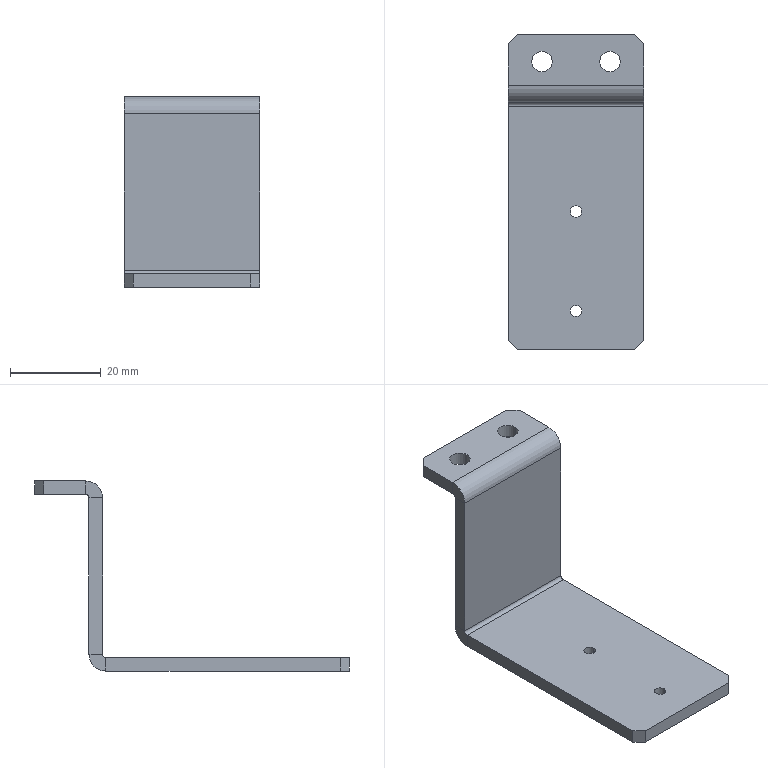Component | SolidWorks | SFTJ-07-DragChainBracket-1 | 1 solid | 34 faces | box 30 x 69.5 x 42 mm | volume 9443 mm3 | plane 22 | cylinder 12 | commonest cylinder face diameters 4.5 x4 2.5 x4 1.473 x2 7.473 x2 | material 201 Annealed Stainless Steel (SS)
STEP:
#1=COLOUR_RGB('',0.7922,0.8196,0.9333);
#2=FILL_AREA_STYLE_COLOUR('',#1);
#3=FILL_AREA_STYLE('',(#2));
#4=SURFACE_STYLE_FILL_AREA(#3);
#5=SURFACE_SIDE_STYLE('',(#4));
#6=SURFACE_STYLE_USAGE(.BOTH.,#5);
#7=PRESENTATION_STYLE_ASSIGNMENT((#6));
#8=CARTESIAN_POINT('',(-8.868,1.839,-2.615));
#9=VERTEX_POINT('',#8);
#10=CARTESIAN_POINT('',(-9.046,1.839,-2.615));
#11=VERTEX_POINT('',#10);
#12=CARTESIAN_POINT('',(-8.957,1.839,-2.615));
#13=DIRECTION('',(-0.,-0.,-1.));
#14=DIRECTION('',(-1.,0.,0.));
#15=AXIS2_PLACEMENT_3D('',#12,#13,#14);
#16=CIRCLE('',#15,0.08858);
#17=EDGE_CURVE('',#9,#11,#16,.T.);
#18=ORIENTED_EDGE('',*,*,#17,.F.);
#19=CARTESIAN_POINT('',(-8.868,1.839,-2.733));
#20=VERTEX_POINT('',#19);
#21=CARTESIAN_POINT('',(-8.868,1.839,-2.733));
#22=DIRECTION('',(-0.,-0.,-1.));
#23=VECTOR('',#22,39.37);
#24=LINE('',#21,#23);
#25=EDGE_CURVE('',#9,#20,#24,.T.);
#26=ORIENTED_EDGE('',*,*,#25,.T.);
#27=CARTESIAN_POINT('',(-9.046,1.839,-2.733));
#28=VERTEX_POINT('',#27);
#29=CARTESIAN_POINT('',(-8.957,1.839,-2.733));
#30=DIRECTION('',(-0.,-0.,-1.));
#31=DIRECTION('',(-1.,0.,0.));
#32=AXIS2_PLACEMENT_3D('',#29,#30,#31);
#33=CIRCLE('',#32,0.08858);
#34=EDGE_CURVE('',#20,#28,#33,.T.);
#35=ORIENTED_EDGE('',*,*,#34,.T.);
#36=CARTESIAN_POINT('',(-9.046,1.839,-2.733));
#37=DIRECTION('',(-0.,-0.,-1.));
#38=VECTOR('',#37,39.37);
#39=LINE('',#36,#38);
#40=EDGE_CURVE('',#11,#28,#39,.T.);
#41=ORIENTED_EDGE('',*,*,#40,.F.);
#42=EDGE_LOOP('',(#18,#26,#35,#41));
#43=FACE_OUTER_BOUND('',#42,.T.);
#44=CARTESIAN_POINT('',(-8.957,1.839,-2.733));
#45=DIRECTION('',(-0.,-0.,-1.));
#46=DIRECTION('',(-1.,0.,0.));
#47=AXIS2_PLACEMENT_3D('',#44,#45,#46);
#48=CYLINDRICAL_SURFACE('',#47,0.08858);
#49=ADVANCED_FACE('',(#43),#48,.F.);
#50=CARTESIAN_POINT('',(-9.459,1.839,-2.615));
#51=VERTEX_POINT('',#50);
#52=CARTESIAN_POINT('',(-9.636,1.839,-2.615));
#53=VERTEX_POINT('',#52);
#54=CARTESIAN_POINT('',(-9.548,1.839,-2.615));
#55=DIRECTION('',(-0.,-0.,-1.));
#56=DIRECTION('',(-1.,0.,0.));
#57=AXIS2_PLACEMENT_3D('',#54,#55,#56);
#58=CIRCLE('',#57,0.08858);
#59=EDGE_CURVE('',#51,#53,#58,.T.);
#60=ORIENTED_EDGE('',*,*,#59,.F.);
#61=CARTESIAN_POINT('',(-9.459,1.839,-2.733));
#62=VERTEX_POINT('',#61);
#63=CARTESIAN_POINT('',(-9.459,1.839,-2.733));
#64=DIRECTION('',(-0.,-0.,-1.));
#65=VECTOR('',#64,39.37);
#66=LINE('',#63,#65);
#67=EDGE_CURVE('',#51,#62,#66,.T.);
#68=ORIENTED_EDGE('',*,*,#67,.T.);
#69=CARTESIAN_POINT('',(-9.636,1.839,-2.733));
#70=VERTEX_POINT('',#69);
#71=CARTESIAN_POINT('',(-9.548,1.839,-2.733));
#72=DIRECTION('',(-0.,-0.,-1.));
#73=DIRECTION('',(-1.,0.,0.));
#74=AXIS2_PLACEMENT_3D('',#71,#72,#73);
#75=CIRCLE('',#74,0.08858);
#76=EDGE_CURVE('',#62,#70,#75,.T.);
#77=ORIENTED_EDGE('',*,*,#76,.T.);
#78=CARTESIAN_POINT('',(-9.636,1.839,-2.733));
#79=DIRECTION('',(-0.,-0.,-1.));
#80=VECTOR('',#79,39.37);
#81=LINE('',#78,#80);
#82=EDGE_CURVE('',#53,#70,#81,.T.);
#83=ORIENTED_EDGE('',*,*,#82,.F.);
#84=EDGE_LOOP('',(#60,#68,#77,#83));
#85=FACE_OUTER_BOUND('',#84,.T.);
#86=CARTESIAN_POINT('',(-9.548,1.839,-2.733));
#87=DIRECTION('',(-0.,-0.,-1.));
#88=DIRECTION('',(-1.,0.,0.));
#89=AXIS2_PLACEMENT_3D('',#86,#87,#88);
#90=CYLINDRICAL_SURFACE('',#89,0.08858);
#91=ADVANCED_FACE('',(#85),#90,.F.);
#92=CARTESIAN_POINT('',(-9.302,-0.326,-4.15));
#93=VERTEX_POINT('',#92);
#94=CARTESIAN_POINT('',(-9.203,-0.326,-4.15));
#95=VERTEX_POINT('',#94);
#96=CARTESIAN_POINT('',(-9.252,-0.326,-4.15));
#97=DIRECTION('',(0.,0.,1.));
#98=DIRECTION('',(0.,1.,0.));
#99=AXIS2_PLACEMENT_3D('',#96,#97,#98);
#100=CIRCLE('',#99,0.04921);
#101=EDGE_CURVE('',#93,#95,#100,.T.);
#102=ORIENTED_EDGE('',*,*,#101,.T.);
#103=CARTESIAN_POINT('',(-9.203,-0.326,-4.268));
#104=VERTEX_POINT('',#103);
#105=CARTESIAN_POINT('',(-9.203,-0.326,-4.268));
#106=DIRECTION('',(-0.,-0.,-1.));
#107=VECTOR('',#106,39.37);
#108=LINE('',#105,#107);
#109=EDGE_CURVE('',#95,#104,#108,.T.);
#110=ORIENTED_EDGE('',*,*,#109,.T.);
#111=CARTESIAN_POINT('',(-9.302,-0.326,-4.268));
#112=VERTEX_POINT('',#111);
#113=CARTESIAN_POINT('',(-9.252,-0.326,-4.268));
#114=DIRECTION('',(-0.,-0.,-1.));
#115=DIRECTION('',(-1.,0.,0.));
#116=AXIS2_PLACEMENT_3D('',#113,#114,#115);
#117=CIRCLE('',#116,0.04921);
#118=EDGE_CURVE('',#104,#112,#117,.T.);
#119=ORIENTED_EDGE('',*,*,#118,.T.);
#120=CARTESIAN_POINT('',(-9.302,-0.326,-4.268));
#121=DIRECTION('',(-0.,-0.,-1.));
#122=VECTOR('',#121,39.37);
#123=LINE('',#120,#122);
#124=EDGE_CURVE('',#93,#112,#123,.T.);
#125=ORIENTED_EDGE('',*,*,#124,.F.);
#126=EDGE_LOOP('',(#102,#110,#119,#125));
#127=FACE_OUTER_BOUND('',#126,.T.);
#128=CARTESIAN_POINT('',(-9.252,-0.326,-4.268));
#129=DIRECTION('',(-0.,-0.,-1.));
#130=DIRECTION('',(-1.,0.,0.));
#131=AXIS2_PLACEMENT_3D('',#128,#129,#130);
#132=CYLINDRICAL_SURFACE('',#131,0.04921);
#133=ADVANCED_FACE('',(#127),#132,.F.);
#134=CARTESIAN_POINT('',(-9.302,0.5402,-4.15));
#135=VERTEX_POINT('',#134);
#136=CARTESIAN_POINT('',(-9.203,0.5402,-4.15));
#137=VERTEX_POINT('',#136);
#138=CARTESIAN_POINT('',(-9.252,0.5402,-4.15));
#139=DIRECTION('',(0.,0.,1.));
#140=DIRECTION('',(0.,1.,0.));
#141=AXIS2_PLACEMENT_3D('',#138,#139,#140);
#142=CIRCLE('',#141,0.04921);
#143=EDGE_CURVE('',#135,#137,#142,.T.);
#144=ORIENTED_EDGE('',*,*,#143,.T.);
#145=CARTESIAN_POINT('',(-9.203,0.5402,-4.268));
#146=VERTEX_POINT('',#145);
#147=CARTESIAN_POINT('',(-9.203,0.5402,-4.268));
#148=DIRECTION('',(-0.,-0.,-1.));
#149=VECTOR('',#148,39.37);
#150=LINE('',#147,#149);
#151=EDGE_CURVE('',#137,#146,#150,.T.);
#152=ORIENTED_EDGE('',*,*,#151,.T.);
#153=CARTESIAN_POINT('',(-9.302,0.5402,-4.268));
#154=VERTEX_POINT('',#153);
#155=CARTESIAN_POINT('',(-9.252,0.5402,-4.268));
#156=DIRECTION('',(-0.,-0.,-1.));
#157=DIRECTION('',(-1.,0.,0.));
#158=AXIS2_PLACEMENT_3D('',#155,#156,#157);
#159=CIRCLE('',#158,0.04921);
#160=EDGE_CURVE('',#146,#154,#159,.T.);
#161=ORIENTED_EDGE('',*,*,#160,.T.);
#162=CARTESIAN_POINT('',(-9.302,0.5402,-4.268));
#163=DIRECTION('',(-0.,-0.,-1.));
#164=VECTOR('',#163,39.37);
#165=LINE('',#162,#164);
#166=EDGE_CURVE('',#135,#154,#165,.T.);
#167=ORIENTED_EDGE('',*,*,#166,.F.);
#168=EDGE_LOOP('',(#144,#152,#161,#167));
#169=FACE_OUTER_BOUND('',#168,.T.);
#170=CARTESIAN_POINT('',(-9.252,0.5402,-4.268));
#171=DIRECTION('',(-0.,-0.,-1.));
#172=DIRECTION('',(-1.,0.,0.));
#173=AXIS2_PLACEMENT_3D('',#170,#171,#172);
#174=CYLINDRICAL_SURFACE('',#173,0.04921);
#175=ADVANCED_FACE('',(#169),#174,.F.);
#176=CARTESIAN_POINT('',(-9.843,1.456,-4.15));
#177=VERTEX_POINT('',#176);
#178=CARTESIAN_POINT('',(-9.843,1.456,-4.268));
#179=VERTEX_POINT('',#178);
#180=CARTESIAN_POINT('',(-9.843,1.456,-4.15));
#181=DIRECTION('',(-0.,-0.,-1.));
#182=VECTOR('',#181,39.37);
#183=LINE('',#180,#182);
#184=EDGE_CURVE('',#177,#179,#183,.T.);
#185=ORIENTED_EDGE('',*,*,#184,.F.);
#186=CARTESIAN_POINT('',(-9.843,1.485,-4.121));
#187=VERTEX_POINT('',#186);
#188=CARTESIAN_POINT('',(-9.843,1.456,-4.121));
#189=DIRECTION('',(-1.,0.,0.));
#190=DIRECTION('',(0.,1.,0.));
#191=AXIS2_PLACEMENT_3D('',#188,#189,#190);
#192=CIRCLE('',#191,0.029);
#193=EDGE_CURVE('',#187,#177,#192,.T.);
#194=ORIENTED_EDGE('',*,*,#193,.F.);
#195=CARTESIAN_POINT('',(-9.843,1.603,-4.121));
#196=VERTEX_POINT('',#195);
#197=CARTESIAN_POINT('',(-9.843,1.603,-4.121));
#198=DIRECTION('',(-0.,-1.,0.));
#199=VECTOR('',#198,39.37);
#200=LINE('',#197,#199);
#201=EDGE_CURVE('',#196,#187,#200,.T.);
#202=ORIENTED_EDGE('',*,*,#201,.F.);
#203=CARTESIAN_POINT('',(-9.843,1.456,-4.121));
#204=DIRECTION('',(-1.,0.,0.));
#205=DIRECTION('',(0.,1.,0.));
#206=AXIS2_PLACEMENT_3D('',#203,#204,#205);
#207=CIRCLE('',#206,0.1471);
#208=EDGE_CURVE('',#196,#179,#207,.T.);
#209=ORIENTED_EDGE('',*,*,#208,.T.);
#210=EDGE_LOOP('',(#185,#194,#202,#209));
#211=FACE_OUTER_BOUND('',#210,.T.);
#212=CARTESIAN_POINT('',(-9.843,1.456,-4.15));
#213=DIRECTION('',(-1.,0.,0.));
#214=DIRECTION('',(0.,1.,-0.));
#215=AXIS2_PLACEMENT_3D('',#212,#213,#214);
#216=PLANE('',#215);
#217=ADVANCED_FACE('',(#211),#216,.T.);
#218=CARTESIAN_POINT('',(-9.843,-0.5819,-4.268));
#219=VERTEX_POINT('',#218);
#220=CARTESIAN_POINT('',(-9.843,1.485,-4.268));
#221=DIRECTION('',(-0.,-1.,0.));
#222=VECTOR('',#221,39.37);
#223=LINE('',#220,#222);
#224=EDGE_CURVE('',#179,#219,#223,.T.);
#225=ORIENTED_EDGE('',*,*,#224,.T.);
#226=CARTESIAN_POINT('',(-9.843,-0.5819,-4.15));
#227=VERTEX_POINT('',#226);
#228=CARTESIAN_POINT('',(-9.843,-0.5819,-4.121));
#229=DIRECTION('',(0.,0.,1.));
#230=VECTOR('',#229,39.37);
#231=LINE('',#228,#230);
#232=EDGE_CURVE('',#219,#227,#231,.T.);
#233=ORIENTED_EDGE('',*,*,#232,.T.);
#234=CARTESIAN_POINT('',(-9.843,1.485,-4.15));
#235=DIRECTION('',(-0.,-1.,0.));
#236=VECTOR('',#235,39.37);
#237=LINE('',#234,#236);
#238=EDGE_CURVE('',#177,#227,#237,.T.);
#239=ORIENTED_EDGE('',*,*,#238,.F.);
#240=ORIENTED_EDGE('',*,*,#184,.T.);
#241=EDGE_LOOP('',(#225,#233,#239,#240));
#242=FACE_OUTER_BOUND('',#241,.T.);
#243=CARTESIAN_POINT('',(-9.843,1.603,-4.121));
#244=DIRECTION('',(-1.,0.,0.));
#245=DIRECTION('',(0.,1.,-0.));
#246=AXIS2_PLACEMENT_3D('',#243,#244,#245);
#247=PLANE('',#246);
#248=ADVANCED_FACE('',(#242),#247,.T.);
#249=CARTESIAN_POINT('',(-8.662,1.485,-4.121));
#250=VERTEX_POINT('',#249);
#251=CARTESIAN_POINT('',(-8.662,1.603,-4.121));
#252=VERTEX_POINT('',#251);
#253=CARTESIAN_POINT('',(-8.662,1.485,-4.121));
#254=DIRECTION('',(0.,1.,-0.));
#255=VECTOR('',#254,39.37);
#256=LINE('',#253,#255);
#257=EDGE_CURVE('',#250,#252,#256,.T.);
#258=ORIENTED_EDGE('',*,*,#257,.F.);
#259=CARTESIAN_POINT('',(-8.662,1.456,-4.15));
#260=VERTEX_POINT('',#259);
#261=CARTESIAN_POINT('',(-8.662,1.456,-4.121));
#262=DIRECTION('',(-1.,0.,0.));
#263=DIRECTION('',(0.,1.,0.));
#264=AXIS2_PLACEMENT_3D('',#261,#262,#263);
#265=CIRCLE('',#264,0.029);
#266=EDGE_CURVE('',#250,#260,#265,.T.);
#267=ORIENTED_EDGE('',*,*,#266,.T.);
#268=CARTESIAN_POINT('',(-8.662,1.456,-4.268));
#269=VERTEX_POINT('',#268);
#270=CARTESIAN_POINT('',(-8.662,1.456,-4.268));
#271=DIRECTION('',(0.,0.,1.));
#272=VECTOR('',#271,39.37);
#273=LINE('',#270,#272);
#274=EDGE_CURVE('',#269,#260,#273,.T.);
#275=ORIENTED_EDGE('',*,*,#274,.F.);
#276=CARTESIAN_POINT('',(-8.662,1.456,-4.121));
#277=DIRECTION('',(-1.,0.,0.));
#278=DIRECTION('',(0.,1.,0.));
#279=AXIS2_PLACEMENT_3D('',#276,#277,#278);
#280=CIRCLE('',#279,0.1471);
#281=EDGE_CURVE('',#252,#269,#280,.T.);
#282=ORIENTED_EDGE('',*,*,#281,.F.);
#283=EDGE_LOOP('',(#258,#267,#275,#282));
#284=FACE_OUTER_BOUND('',#283,.T.);
#285=CARTESIAN_POINT('',(-8.662,1.485,-4.121));
#286=DIRECTION('',(1.,-0.,-0.));
#287=DIRECTION('',(-0.,-1.,0.));
#288=AXIS2_PLACEMENT_3D('',#285,#286,#287);
#289=PLANE('',#288);
#290=ADVANCED_FACE('',(#284),#289,.T.);
#291=CARTESIAN_POINT('',(-8.662,1.485,-2.762));
#292=VERTEX_POINT('',#291);
#293=CARTESIAN_POINT('',(-8.662,1.485,-2.615));
#294=DIRECTION('',(-0.,-0.,-1.));
#295=VECTOR('',#294,39.37);
#296=LINE('',#293,#295);
#297=EDGE_CURVE('',#292,#250,#296,.T.);
#298=ORIENTED_EDGE('',*,*,#297,.T.);
#299=ORIENTED_EDGE('',*,*,#257,.T.);
#300=CARTESIAN_POINT('',(-8.662,1.603,-2.762));
#301=VERTEX_POINT('',#300);
#302=CARTESIAN_POINT('',(-8.662,1.603,-2.615));
#303=DIRECTION('',(-0.,-0.,-1.));
#304=VECTOR('',#303,39.37);
#305=LINE('',#302,#304);
#306=EDGE_CURVE('',#301,#252,#305,.T.);
#307=ORIENTED_EDGE('',*,*,#306,.F.);
#308=CARTESIAN_POINT('',(-8.662,1.603,-2.762));
#309=DIRECTION('',(-0.,-1.,0.));
#310=VECTOR('',#309,39.37);
#311=LINE('',#308,#310);
#312=EDGE_CURVE('',#301,#292,#311,.T.);
#313=ORIENTED_EDGE('',*,*,#312,.T.);
#314=EDGE_LOOP('',(#298,#299,#307,#313));
#315=FACE_OUTER_BOUND('',#314,.T.);
#316=CARTESIAN_POINT('',(-8.662,1.456,-4.268));
#317=DIRECTION('',(1.,-0.,-0.));
#318=DIRECTION('',(-0.,-1.,0.));
#319=AXIS2_PLACEMENT_3D('',#316,#317,#318);
#320=PLANE('',#319);
#321=ADVANCED_FACE('',(#315),#320,.T.);
#322=CARTESIAN_POINT('',(-9.843,1.485,-2.762));
#323=VERTEX_POINT('',#322);
#324=CARTESIAN_POINT('',(-9.843,1.603,-2.762));
#325=VERTEX_POINT('',#324);
#326=CARTESIAN_POINT('',(-9.843,1.485,-2.762));
#327=DIRECTION('',(0.,1.,-0.));
#328=VECTOR('',#327,39.37);
#329=LINE('',#326,#328);
#330=EDGE_CURVE('',#323,#325,#329,.T.);
#331=ORIENTED_EDGE('',*,*,#330,.F.);
#332=CARTESIAN_POINT('',(-9.843,1.632,-2.615));
#333=VERTEX_POINT('',#332);
#334=CARTESIAN_POINT('',(-9.843,1.632,-2.762));
#335=DIRECTION('',(1.,-0.,-0.));
#336=DIRECTION('',(0.,-1.,0.));
#337=AXIS2_PLACEMENT_3D('',#334,#335,#336);
#338=CIRCLE('',#337,0.1471);
#339=EDGE_CURVE('',#333,#323,#338,.T.);
#340=ORIENTED_EDGE('',*,*,#339,.F.);
#341=CARTESIAN_POINT('',(-9.843,1.632,-2.733));
#342=VERTEX_POINT('',#341);
#343=CARTESIAN_POINT('',(-9.843,1.632,-2.733));
#344=DIRECTION('',(0.,0.,1.));
#345=VECTOR('',#344,39.37);
#346=LINE('',#343,#345);
#347=EDGE_CURVE('',#342,#333,#346,.T.);
#348=ORIENTED_EDGE('',*,*,#347,.F.);
#349=CARTESIAN_POINT('',(-9.843,1.632,-2.762));
#350=DIRECTION('',(1.,-0.,-0.));
#351=DIRECTION('',(0.,1.,0.));
#352=AXIS2_PLACEMENT_3D('',#349,#350,#351);
#353=CIRCLE('',#352,0.029);
#354=EDGE_CURVE('',#342,#325,#353,.T.);
#355=ORIENTED_EDGE('',*,*,#354,.T.);
#356=EDGE_LOOP('',(#331,#340,#348,#355));
#357=FACE_OUTER_BOUND('',#356,.T.);
#358=CARTESIAN_POINT('',(-9.843,1.485,-2.762));
#359=DIRECTION('',(-1.,0.,0.));
#360=DIRECTION('',(0.,1.,-0.));
#361=AXIS2_PLACEMENT_3D('',#358,#359,#360);
#362=PLANE('',#361);
#363=ADVANCED_FACE('',(#357),#362,.T.);
#364=CARTESIAN_POINT('',(-9.843,1.485,-2.615));
#365=DIRECTION('',(-0.,-0.,-1.));
#366=VECTOR('',#365,39.37);
#367=LINE('',#364,#366);
#368=EDGE_CURVE('',#323,#187,#367,.T.);
#369=ORIENTED_EDGE('',*,*,#368,.F.);
#370=ORIENTED_EDGE('',*,*,#330,.T.);
#371=CARTESIAN_POINT('',(-9.843,1.603,-2.615));
#372=DIRECTION('',(-0.,-0.,-1.));
#373=VECTOR('',#372,39.37);
#374=LINE('',#371,#373);
#375=EDGE_CURVE('',#325,#196,#374,.T.);
#376=ORIENTED_EDGE('',*,*,#375,.T.);
#377=ORIENTED_EDGE('',*,*,#201,.T.);
#378=EDGE_LOOP('',(#369,#370,#376,#377));
#379=FACE_OUTER_BOUND('',#378,.T.);
#380=CARTESIAN_POINT('',(-9.843,1.632,-2.733));
#381=DIRECTION('',(-1.,0.,0.));
#382=DIRECTION('',(0.,1.,-0.));
#383=AXIS2_PLACEMENT_3D('',#380,#381,#382);
#384=PLANE('',#383);
#385=ADVANCED_FACE('',(#379),#384,.T.);
#386=CARTESIAN_POINT('',(-8.662,1.632,-2.615));
#387=VERTEX_POINT('',#386);
#388=CARTESIAN_POINT('',(-8.662,1.632,-2.733));
#389=VERTEX_POINT('',#388);
#390=CARTESIAN_POINT('',(-8.662,1.632,-2.615));
#391=DIRECTION('',(-0.,-0.,-1.));
#392=VECTOR('',#391,39.37);
#393=LINE('',#390,#392);
#394=EDGE_CURVE('',#387,#389,#393,.T.);
#395=ORIENTED_EDGE('',*,*,#394,.F.);
#396=CARTESIAN_POINT('',(-8.662,1.632,-2.762));
#397=DIRECTION('',(1.,-0.,-0.));
#398=DIRECTION('',(0.,-1.,0.));
#399=AXIS2_PLACEMENT_3D('',#396,#397,#398);
#400=CIRCLE('',#399,0.1471);
#401=EDGE_CURVE('',#387,#292,#400,.T.);
#402=ORIENTED_EDGE('',*,*,#401,.T.);
#403=ORIENTED_EDGE('',*,*,#312,.F.);
#404=CARTESIAN_POINT('',(-8.662,1.632,-2.762));
#405=DIRECTION('',(1.,-0.,-0.));
#406=DIRECTION('',(0.,1.,0.));
#407=AXIS2_PLACEMENT_3D('',#404,#405,#406);
#408=CIRCLE('',#407,0.029);
#409=EDGE_CURVE('',#389,#301,#408,.T.);
#410=ORIENTED_EDGE('',*,*,#409,.F.);
#411=EDGE_LOOP('',(#395,#402,#403,#410));
#412=FACE_OUTER_BOUND('',#411,.T.);
#413=CARTESIAN_POINT('',(-8.662,1.632,-2.615));
#414=DIRECTION('',(1.,-0.,-0.));
#415=DIRECTION('',(-0.,-1.,0.));
#416=AXIS2_PLACEMENT_3D('',#413,#414,#415);
#417=PLANE('',#416);
#418=ADVANCED_FACE('',(#412),#417,.T.);
#419=CARTESIAN_POINT('',(-8.662,1.997,-2.733));
#420=VERTEX_POINT('',#419);
#421=CARTESIAN_POINT('',(-8.662,1.485,-2.733));
#422=DIRECTION('',(-0.,-1.,0.));
#423=VECTOR('',#422,39.37);
#424=LINE('',#421,#423);
#425=EDGE_CURVE('',#420,#389,#424,.T.);
#426=ORIENTED_EDGE('',*,*,#425,.F.);
#427=CARTESIAN_POINT('',(-8.662,1.997,-2.615));
#428=VERTEX_POINT('',#427);
#429=CARTESIAN_POINT('',(-8.662,1.997,-2.762));
#430=DIRECTION('',(0.,0.,1.));
#431=VECTOR('',#430,39.37);
#432=LINE('',#429,#431);
#433=EDGE_CURVE('',#420,#428,#432,.T.);
#434=ORIENTED_EDGE('',*,*,#433,.T.);
#435=CARTESIAN_POINT('',(-8.662,1.485,-2.615));
#436=DIRECTION('',(-0.,-1.,0.));
#437=VECTOR('',#436,39.37);
#438=LINE('',#435,#437);
#439=EDGE_CURVE('',#428,#387,#438,.T.);
#440=ORIENTED_EDGE('',*,*,#439,.T.);
#441=ORIENTED_EDGE('',*,*,#394,.T.);
#442=EDGE_LOOP('',(#426,#434,#440,#441));
#443=FACE_OUTER_BOUND('',#442,.T.);
#444=CARTESIAN_POINT('',(-8.662,1.603,-2.762));
#445=DIRECTION('',(1.,-0.,-0.));
#446=DIRECTION('',(-0.,-1.,0.));
#447=AXIS2_PLACEMENT_3D('',#444,#445,#446);
#448=PLANE('',#447);
#449=ADVANCED_FACE('',(#443),#448,.T.);
#450=CARTESIAN_POINT('',(-9.252,-0.326,-4.268));
#451=DIRECTION('',(-0.,-0.,-1.));
#452=DIRECTION('',(-1.,0.,0.));
#453=AXIS2_PLACEMENT_3D('',#450,#451,#452);
#454=CIRCLE('',#453,0.04921);
#455=EDGE_CURVE('',#112,#104,#454,.T.);
#456=ORIENTED_EDGE('',*,*,#455,.F.);
#457=ORIENTED_EDGE('',*,*,#118,.F.);
#458=EDGE_LOOP('',(#456,#457));
#459=FACE_BOUND('',#458,.T.);
#460=CARTESIAN_POINT('',(-9.252,0.5402,-4.268));
#461=DIRECTION('',(-0.,-0.,-1.));
#462=DIRECTION('',(-1.,0.,0.));
#463=AXIS2_PLACEMENT_3D('',#460,#461,#462);
#464=CIRCLE('',#463,0.04921);
#465=EDGE_CURVE('',#154,#146,#464,.T.);
#466=ORIENTED_EDGE('',*,*,#465,.F.);
#467=ORIENTED_EDGE('',*,*,#160,.F.);
#468=EDGE_LOOP('',(#466,#467));
#469=FACE_BOUND('',#468,.T.);
#470=CARTESIAN_POINT('',(-8.662,-0.5819,-4.268));
#471=VERTEX_POINT('',#470);
#472=CARTESIAN_POINT('',(-8.662,1.485,-4.268));
#473=DIRECTION('',(-0.,-1.,0.));
#474=VECTOR('',#473,39.37);
#475=LINE('',#472,#474);
#476=EDGE_CURVE('',#269,#471,#475,.T.);
#477=ORIENTED_EDGE('',*,*,#476,.T.);
#478=CARTESIAN_POINT('',(-8.741,-0.6606,-4.268));
#479=VERTEX_POINT('',#478);
#480=CARTESIAN_POINT('',(-8.662,-0.5819,-4.268));
#481=DIRECTION('',(-0.7071,-0.7071,0.));
#482=VECTOR('',#481,39.37);
#483=LINE('',#480,#482);
#484=EDGE_CURVE('',#471,#479,#483,.T.);
#485=ORIENTED_EDGE('',*,*,#484,.T.);
#486=CARTESIAN_POINT('',(-9.764,-0.6606,-4.268));
#487=VERTEX_POINT('',#486);
#488=CARTESIAN_POINT('',(-9.843,-0.6606,-4.268));
#489=DIRECTION('',(1.,-0.,-0.));
#490=VECTOR('',#489,39.37);
#491=LINE('',#488,#490);
#492=EDGE_CURVE('',#487,#479,#491,.T.);
#493=ORIENTED_EDGE('',*,*,#492,.F.);
#494=CARTESIAN_POINT('',(-9.764,-0.6606,-4.268));
#495=DIRECTION('',(-0.7071,0.7071,-0.));
#496=VECTOR('',#495,39.37);
#497=LINE('',#494,#496);
#498=EDGE_CURVE('',#487,#219,#497,.T.);
#499=ORIENTED_EDGE('',*,*,#498,.T.);
#500=ORIENTED_EDGE('',*,*,#224,.F.);
#501=CARTESIAN_POINT('',(-9.843,1.456,-4.268));
#502=DIRECTION('',(1.,-0.,-0.));
#503=VECTOR('',#502,39.37);
#504=LINE('',#501,#503);
#505=EDGE_CURVE('',#179,#269,#504,.T.);
#506=ORIENTED_EDGE('',*,*,#505,.T.);
#507=EDGE_LOOP('',(#477,#485,#493,#499,#500,#506));
#508=FACE_OUTER_BOUND('',#507,.T.);
#509=CARTESIAN_POINT('',(-9.843,1.485,-4.268));
#510=DIRECTION('',(0.,0.,1.));
#511=DIRECTION('',(0.,1.,-0.));
#512=AXIS2_PLACEMENT_3D('',#509,#510,#511);
#513=PLANE('',#512);
#514=ADVANCED_FACE('',(#459,#469,#508),#513,.F.);
#515=ORIENTED_EDGE('',*,*,#492,.T.);
#516=CARTESIAN_POINT('',(-8.741,-0.6606,-4.15));
#517=VERTEX_POINT('',#516);
#518=CARTESIAN_POINT('',(-8.741,-0.6606,-4.15));
#519=DIRECTION('',(0.,0.,1.));
#520=VECTOR('',#519,39.37);
#521=LINE('',#518,#520);
#522=EDGE_CURVE('',#479,#517,#521,.T.);
#523=ORIENTED_EDGE('',*,*,#522,.T.);
#524=CARTESIAN_POINT('',(-9.764,-0.6606,-4.15));
#525=VERTEX_POINT('',#524);
#526=CARTESIAN_POINT('',(-9.843,-0.6606,-4.15));
#527=DIRECTION('',(1.,-0.,-0.));
#528=VECTOR('',#527,39.37);
#529=LINE('',#526,#528);
#530=EDGE_CURVE('',#525,#517,#529,.T.);
#531=ORIENTED_EDGE('',*,*,#530,.F.);
#532=CARTESIAN_POINT('',(-9.764,-0.6606,-4.15));
#533=DIRECTION('',(-0.,-0.,-1.));
#534=VECTOR('',#533,39.37);
#535=LINE('',#532,#534);
#536=EDGE_CURVE('',#525,#487,#535,.T.);
#537=ORIENTED_EDGE('',*,*,#536,.T.);
#538=EDGE_LOOP('',(#515,#523,#531,#537));
#539=FACE_OUTER_BOUND('',#538,.T.);
#540=CARTESIAN_POINT('',(-9.843,-0.6606,-4.15));
#541=DIRECTION('',(-0.,-1.,0.));
#542=DIRECTION('',(-1.,0.,0.));
#543=AXIS2_PLACEMENT_3D('',#540,#541,#542);
#544=PLANE('',#543);
#545=ADVANCED_FACE('',(#539),#544,.T.);
#546=ORIENTED_EDGE('',*,*,#101,.F.);
#547=CARTESIAN_POINT('',(-9.252,-0.326,-4.15));
#548=DIRECTION('',(0.,0.,1.));
#549=DIRECTION('',(0.,1.,0.));
#550=AXIS2_PLACEMENT_3D('',#547,#548,#549);
#551=CIRCLE('',#550,0.04921);
#552=EDGE_CURVE('',#95,#93,#551,.T.);
#553=ORIENTED_EDGE('',*,*,#552,.F.);
#554=EDGE_LOOP('',(#546,#553));
#555=FACE_BOUND('',#554,.T.);
#556=ORIENTED_EDGE('',*,*,#143,.F.);
#557=CARTESIAN_POINT('',(-9.252,0.5402,-4.15));
#558=DIRECTION('',(0.,0.,1.));
#559=DIRECTION('',(0.,1.,0.));
#560=AXIS2_PLACEMENT_3D('',#557,#558,#559);
#561=CIRCLE('',#560,0.04921);
#562=EDGE_CURVE('',#137,#135,#561,.T.);
#563=ORIENTED_EDGE('',*,*,#562,.F.);
#564=EDGE_LOOP('',(#556,#563));
#565=FACE_BOUND('',#564,.T.);
#566=ORIENTED_EDGE('',*,*,#530,.T.);
#567=CARTESIAN_POINT('',(-8.662,-0.5819,-4.15));
#568=VERTEX_POINT('',#567);
#569=CARTESIAN_POINT('',(-8.219,-0.139,-4.15));
#570=DIRECTION('',(0.7071,0.7071,-0.));
#571=VECTOR('',#570,39.37);
#572=LINE('',#569,#571);
#573=EDGE_CURVE('',#517,#568,#572,.T.);
#574=ORIENTED_EDGE('',*,*,#573,.T.);
#575=CARTESIAN_POINT('',(-8.662,1.485,-4.15));
#576=DIRECTION('',(-0.,-1.,0.));
#577=VECTOR('',#576,39.37);
#578=LINE('',#575,#577);
#579=EDGE_CURVE('',#260,#568,#578,.T.);
#580=ORIENTED_EDGE('',*,*,#579,.F.);
#581=CARTESIAN_POINT('',(-9.843,1.456,-4.15));
#582=DIRECTION('',(1.,-0.,-0.));
#583=VECTOR('',#582,39.37);
#584=LINE('',#581,#583);
#585=EDGE_CURVE('',#177,#260,#584,.T.);
#586=ORIENTED_EDGE('',*,*,#585,.F.);
#587=ORIENTED_EDGE('',*,*,#238,.T.);
#588=CARTESIAN_POINT('',(-10.876,0.4516,-4.15));
#589=DIRECTION('',(0.7071,-0.7071,0.));
#590=VECTOR('',#589,39.37);
#591=LINE('',#588,#590);
#592=EDGE_CURVE('',#227,#525,#591,.T.);
#593=ORIENTED_EDGE('',*,*,#592,.T.);
#594=EDGE_LOOP('',(#566,#574,#580,#586,#587,#593));
#595=FACE_OUTER_BOUND('',#594,.T.);
#596=CARTESIAN_POINT('',(-9.843,1.485,-4.15));
#597=DIRECTION('',(0.,0.,1.));
#598=DIRECTION('',(0.,1.,-0.));
#599=AXIS2_PLACEMENT_3D('',#596,#597,#598);
#600=PLANE('',#599);
#601=ADVANCED_FACE('',(#555,#565,#595),#600,.T.);
#602=ORIENTED_EDGE('',*,*,#266,.F.);
#603=CARTESIAN_POINT('',(-9.843,1.485,-4.121));
#604=DIRECTION('',(1.,-0.,-0.));
#605=VECTOR('',#604,39.37);
#606=LINE('',#603,#605);
#607=EDGE_CURVE('',#187,#250,#606,.T.);
#608=ORIENTED_EDGE('',*,*,#607,.F.);
#609=ORIENTED_EDGE('',*,*,#193,.T.);
#610=ORIENTED_EDGE('',*,*,#585,.T.);
#611=EDGE_LOOP('',(#602,#608,#609,#610));
#612=FACE_OUTER_BOUND('',#611,.T.);
#613=CARTESIAN_POINT('',(-9.843,1.456,-4.121));
#614=DIRECTION('',(1.,-0.,-0.));
#615=DIRECTION('',(0.,-1.,0.));
#616=AXIS2_PLACEMENT_3D('',#613,#614,#615);
#617=CYLINDRICAL_SURFACE('',#616,0.029);
#618=ADVANCED_FACE('',(#612),#617,.F.);
#619=ORIENTED_EDGE('',*,*,#297,.F.);
#620=CARTESIAN_POINT('',(-9.843,1.485,-2.762));
#621=DIRECTION('',(1.,-0.,-0.));
#622=VECTOR('',#621,39.37);
#623=LINE('',#620,#622);
#624=EDGE_CURVE('',#323,#292,#623,.T.);
#625=ORIENTED_EDGE('',*,*,#624,.F.);
#626=ORIENTED_EDGE('',*,*,#368,.T.);
#627=ORIENTED_EDGE('',*,*,#607,.T.);
#628=EDGE_LOOP('',(#619,#625,#626,#627));
#629=FACE_OUTER_BOUND('',#628,.T.);
#630=CARTESIAN_POINT('',(-9.843,1.485,-2.615));
#631=DIRECTION('',(-0.,-1.,0.));
#632=DIRECTION('',(-1.,0.,0.));
#633=AXIS2_PLACEMENT_3D('',#630,#631,#632);
#634=PLANE('',#633);
#635=ADVANCED_FACE('',(#629),#634,.T.);
#636=ORIENTED_EDGE('',*,*,#401,.F.);
#637=CARTESIAN_POINT('',(-9.843,1.632,-2.615));
#638=DIRECTION('',(1.,-0.,-0.));
#639=VECTOR('',#638,39.37);
#640=LINE('',#637,#639);
#641=EDGE_CURVE('',#333,#387,#640,.T.);
#642=ORIENTED_EDGE('',*,*,#641,.F.);
#643=ORIENTED_EDGE('',*,*,#339,.T.);
#644=ORIENTED_EDGE('',*,*,#624,.T.);
#645=EDGE_LOOP('',(#636,#642,#643,#644));
#646=FACE_OUTER_BOUND('',#645,.T.);
#647=CARTESIAN_POINT('',(-9.843,1.632,-2.762));
#648=DIRECTION('',(1.,-0.,-0.));
#649=DIRECTION('',(0.,-1.,0.));
#650=AXIS2_PLACEMENT_3D('',#647,#648,#649);
#651=CYLINDRICAL_SURFACE('',#650,0.1471);
#652=ADVANCED_FACE('',(#646),#651,.T.);
#653=CARTESIAN_POINT('',(-8.957,1.839,-2.615));
#654=DIRECTION('',(-0.,-0.,-1.));
#655=DIRECTION('',(-1.,0.,0.));
#656=AXIS2_PLACEMENT_3D('',#653,#654,#655);
#657=CIRCLE('',#656,0.08858);
#658=EDGE_CURVE('',#11,#9,#657,.T.);
#659=ORIENTED_EDGE('',*,*,#658,.T.);
#660=ORIENTED_EDGE('',*,*,#17,.T.);
#661=EDGE_LOOP('',(#659,#660));
#662=FACE_BOUND('',#661,.T.);
#663=CARTESIAN_POINT('',(-9.548,1.839,-2.615));
#664=DIRECTION('',(-0.,-0.,-1.));
#665=DIRECTION('',(-1.,0.,0.));
#666=AXIS2_PLACEMENT_3D('',#663,#664,#665);
#667=CIRCLE('',#666,0.08858);
#668=EDGE_CURVE('',#53,#51,#667,.T.);
#669=ORIENTED_EDGE('',*,*,#668,.T.);
#670=ORIENTED_EDGE('',*,*,#59,.T.);
#671=EDGE_LOOP('',(#669,#670));
#672=FACE_BOUND('',#671,.T.);
#673=ORIENTED_EDGE('',*,*,#439,.F.);
#674=CARTESIAN_POINT('',(-8.741,2.076,-2.615));
#675=VERTEX_POINT('',#674);
#676=CARTESIAN_POINT('',(-8.996,2.332,-2.615));
#677=DIRECTION('',(-0.7071,0.7071,-0.));
#678=VECTOR('',#677,39.37);
#679=LINE('',#676,#678);
#680=EDGE_CURVE('',#428,#675,#679,.T.);
#681=ORIENTED_EDGE('',*,*,#680,.T.);
#682=CARTESIAN_POINT('',(-9.764,2.076,-2.615));
#683=VERTEX_POINT('',#682);
#684=CARTESIAN_POINT('',(-9.843,2.076,-2.615));
#685=DIRECTION('',(1.,-0.,-0.));
#686=VECTOR('',#685,39.37);
#687=LINE('',#684,#686);
#688=EDGE_CURVE('',#683,#675,#687,.T.);
#689=ORIENTED_EDGE('',*,*,#688,.F.);
#690=CARTESIAN_POINT('',(-9.843,1.997,-2.615));
#691=VERTEX_POINT('',#690);
#692=CARTESIAN_POINT('',(-10.099,1.741,-2.615));
#693=DIRECTION('',(-0.7071,-0.7071,0.));
#694=VECTOR('',#693,39.37);
#695=LINE('',#692,#694);
#696=EDGE_CURVE('',#683,#691,#695,.T.);
#697=ORIENTED_EDGE('',*,*,#696,.T.);
#698=CARTESIAN_POINT('',(-9.843,1.485,-2.615));
#699=DIRECTION('',(-0.,-1.,0.));
#700=VECTOR('',#699,39.37);
#701=LINE('',#698,#700);
#702=EDGE_CURVE('',#691,#333,#701,.T.);
#703=ORIENTED_EDGE('',*,*,#702,.T.);
#704=ORIENTED_EDGE('',*,*,#641,.T.);
#705=EDGE_LOOP('',(#673,#681,#689,#697,#703,#704));
#706=FACE_OUTER_BOUND('',#705,.T.);
#707=CARTESIAN_POINT('',(-9.843,1.485,-2.615));
#708=DIRECTION('',(0.,0.,1.));
#709=DIRECTION('',(1.,-0.,-0.));
#710=AXIS2_PLACEMENT_3D('',#707,#708,#709);
#711=PLANE('',#710);
#712=ADVANCED_FACE('',(#662,#672,#706),#711,.T.);
#713=ORIENTED_EDGE('',*,*,#688,.T.);
#714=CARTESIAN_POINT('',(-8.741,2.076,-2.733));
#715=VERTEX_POINT('',#714);
#716=CARTESIAN_POINT('',(-8.741,2.076,-2.733));
#717=DIRECTION('',(-0.,-0.,-1.));
#718=VECTOR('',#717,39.37);
#719=LINE('',#716,#718);
#720=EDGE_CURVE('',#675,#715,#719,.T.);
#721=ORIENTED_EDGE('',*,*,#720,.T.);
#722=CARTESIAN_POINT('',(-9.764,2.076,-2.733));
#723=VERTEX_POINT('',#722);
#724=CARTESIAN_POINT('',(-9.843,2.076,-2.733));
#725=DIRECTION('',(1.,-0.,-0.));
#726=VECTOR('',#725,39.37);
#727=LINE('',#724,#726);
#728=EDGE_CURVE('',#723,#715,#727,.T.);
#729=ORIENTED_EDGE('',*,*,#728,.F.);
#730=CARTESIAN_POINT('',(-9.764,2.076,-2.733));
#731=DIRECTION('',(0.,0.,1.));
#732=VECTOR('',#731,39.37);
#733=LINE('',#730,#732);
#734=EDGE_CURVE('',#723,#683,#733,.T.);
#735=ORIENTED_EDGE('',*,*,#734,.T.);
#736=EDGE_LOOP('',(#713,#721,#729,#735));
#737=FACE_OUTER_BOUND('',#736,.T.);
#738=CARTESIAN_POINT('',(-9.843,2.076,-2.733));
#739=DIRECTION('',(0.,1.,-0.));
#740=DIRECTION('',(1.,-0.,-0.));
#741=AXIS2_PLACEMENT_3D('',#738,#739,#740);
#742=PLANE('',#741);
#743=ADVANCED_FACE('',(#737),#742,.T.);
#744=CARTESIAN_POINT('',(-8.957,1.839,-2.733));
#745=DIRECTION('',(-0.,-0.,-1.));
#746=DIRECTION('',(-1.,0.,0.));
#747=AXIS2_PLACEMENT_3D('',#744,#745,#746);
#748=CIRCLE('',#747,0.08858);
#749=EDGE_CURVE('',#28,#20,#748,.T.);
#750=ORIENTED_EDGE('',*,*,#749,.F.);
#751=ORIENTED_EDGE('',*,*,#34,.F.);
#752=EDGE_LOOP('',(#750,#751));
#753=FACE_BOUND('',#752,.T.);
#754=CARTESIAN_POINT('',(-9.548,1.839,-2.733));
#755=DIRECTION('',(-0.,-0.,-1.));
#756=DIRECTION('',(-1.,0.,0.));
#757=AXIS2_PLACEMENT_3D('',#754,#755,#756);
#758=CIRCLE('',#757,0.08858);
#759=EDGE_CURVE('',#70,#62,#758,.T.);
#760=ORIENTED_EDGE('',*,*,#759,.F.);
#761=ORIENTED_EDGE('',*,*,#76,.F.);
#762=EDGE_LOOP('',(#760,#761));
#763=FACE_BOUND('',#762,.T.);
#764=ORIENTED_EDGE('',*,*,#728,.T.);
#765=CARTESIAN_POINT('',(-8.662,1.997,-2.733));
#766=DIRECTION('',(0.7071,-0.7071,0.));
#767=VECTOR('',#766,39.37);
#768=LINE('',#765,#767);
#769=EDGE_CURVE('',#715,#420,#768,.T.);
#770=ORIENTED_EDGE('',*,*,#769,.T.);
#771=ORIENTED_EDGE('',*,*,#425,.T.);
#772=CARTESIAN_POINT('',(-9.843,1.632,-2.733));
#773=DIRECTION('',(1.,-0.,-0.));
#774=VECTOR('',#773,39.37);
#775=LINE('',#772,#774);
#776=EDGE_CURVE('',#342,#389,#775,.T.);
#777=ORIENTED_EDGE('',*,*,#776,.F.);
#778=CARTESIAN_POINT('',(-9.843,1.997,-2.733));
#779=VERTEX_POINT('',#778);
#780=CARTESIAN_POINT('',(-9.843,1.485,-2.733));
#781=DIRECTION('',(-0.,-1.,0.));
#782=VECTOR('',#781,39.37);
#783=LINE('',#780,#782);
#784=EDGE_CURVE('',#779,#342,#783,.T.);
#785=ORIENTED_EDGE('',*,*,#784,.F.);
#786=CARTESIAN_POINT('',(-9.764,2.076,-2.733));
#787=DIRECTION('',(0.7071,0.7071,-0.));
#788=VECTOR('',#787,39.37);
#789=LINE('',#786,#788);
#790=EDGE_CURVE('',#779,#723,#789,.T.);
#791=ORIENTED_EDGE('',*,*,#790,.T.);
#792=EDGE_LOOP('',(#764,#770,#771,#777,#785,#791));
#793=FACE_OUTER_BOUND('',#792,.T.);
#794=CARTESIAN_POINT('',(-9.843,1.485,-2.733));
#795=DIRECTION('',(0.,0.,1.));
#796=DIRECTION('',(1.,-0.,-0.));
#797=AXIS2_PLACEMENT_3D('',#794,#795,#796);
#798=PLANE('',#797);
#799=ADVANCED_FACE('',(#753,#763,#793),#798,.F.);
#800=ORIENTED_EDGE('',*,*,#409,.T.);
#801=CARTESIAN_POINT('',(-9.843,1.603,-2.762));
#802=DIRECTION('',(1.,-0.,-0.));
#803=VECTOR('',#802,39.37);
#804=LINE('',#801,#803);
#805=EDGE_CURVE('',#325,#301,#804,.T.);
#806=ORIENTED_EDGE('',*,*,#805,.F.);
#807=ORIENTED_EDGE('',*,*,#354,.F.);
#808=ORIENTED_EDGE('',*,*,#776,.T.);
#809=EDGE_LOOP('',(#800,#806,#807,#808));
#810=FACE_OUTER_BOUND('',#809,.T.);
#811=CARTESIAN_POINT('',(-9.843,1.632,-2.762));
#812=DIRECTION('',(1.,-0.,-0.));
#813=DIRECTION('',(0.,-1.,0.));
#814=AXIS2_PLACEMENT_3D('',#811,#812,#813);
#815=CYLINDRICAL_SURFACE('',#814,0.029);
#816=ADVANCED_FACE('',(#810),#815,.F.);
#817=ORIENTED_EDGE('',*,*,#306,.T.);
#818=CARTESIAN_POINT('',(-9.843,1.603,-4.121));
#819=DIRECTION('',(1.,-0.,-0.));
#820=VECTOR('',#819,39.37);
#821=LINE('',#818,#820);
#822=EDGE_CURVE('',#196,#252,#821,.T.);
#823=ORIENTED_EDGE('',*,*,#822,.F.);
#824=ORIENTED_EDGE('',*,*,#375,.F.);
#825=ORIENTED_EDGE('',*,*,#805,.T.);
#826=EDGE_LOOP('',(#817,#823,#824,#825));
#827=FACE_OUTER_BOUND('',#826,.T.);
#828=CARTESIAN_POINT('',(-9.843,1.603,-2.615));
#829=DIRECTION('',(-0.,-1.,0.));
#830=DIRECTION('',(-1.,0.,0.));
#831=AXIS2_PLACEMENT_3D('',#828,#829,#830);
#832=PLANE('',#831);
#833=ADVANCED_FACE('',(#827),#832,.F.);
#834=ORIENTED_EDGE('',*,*,#281,.T.);
#835=ORIENTED_EDGE('',*,*,#505,.F.);
#836=ORIENTED_EDGE('',*,*,#208,.F.);
#837=ORIENTED_EDGE('',*,*,#822,.T.);
#838=EDGE_LOOP('',(#834,#835,#836,#837));
#839=FACE_OUTER_BOUND('',#838,.T.);
#840=CARTESIAN_POINT('',(-9.843,1.456,-4.121));
#841=DIRECTION('',(1.,-0.,-0.));
#842=DIRECTION('',(0.,-1.,0.));
#843=AXIS2_PLACEMENT_3D('',#840,#841,#842);
#844=CYLINDRICAL_SURFACE('',#843,0.1471);
#845=ADVANCED_FACE('',(#839),#844,.T.);
#846=ORIENTED_EDGE('',*,*,#702,.F.);
#847=CARTESIAN_POINT('',(-9.843,1.997,-4.121));
#848=DIRECTION('',(-0.,-0.,-1.));
#849=VECTOR('',#848,39.37);
#850=LINE('',#847,#849);
#851=EDGE_CURVE('',#691,#779,#850,.T.);
#852=ORIENTED_EDGE('',*,*,#851,.T.);
#853=ORIENTED_EDGE('',*,*,#784,.T.);
#854=ORIENTED_EDGE('',*,*,#347,.T.);
#855=EDGE_LOOP('',(#846,#852,#853,#854));
#856=FACE_OUTER_BOUND('',#855,.T.);
#857=CARTESIAN_POINT('',(-9.843,1.456,-4.121));
#858=DIRECTION('',(-1.,0.,0.));
#859=DIRECTION('',(0.,1.,-0.));
#860=AXIS2_PLACEMENT_3D('',#857,#858,#859);
#861=PLANE('',#860);
#862=ADVANCED_FACE('',(#856),#861,.T.);
#863=ORIENTED_EDGE('',*,*,#579,.T.);
#864=CARTESIAN_POINT('',(-8.662,-0.5819,-4.268));
#865=DIRECTION('',(-0.,-0.,-1.));
#866=VECTOR('',#865,39.37);
#867=LINE('',#864,#866);
#868=EDGE_CURVE('',#568,#471,#867,.T.);
#869=ORIENTED_EDGE('',*,*,#868,.T.);
#870=ORIENTED_EDGE('',*,*,#476,.F.);
#871=ORIENTED_EDGE('',*,*,#274,.T.);
#872=EDGE_LOOP('',(#863,#869,#870,#871));
#873=FACE_OUTER_BOUND('',#872,.T.);
#874=CARTESIAN_POINT('',(-8.662,1.456,-4.121));
#875=DIRECTION('',(-1.,0.,0.));
#876=DIRECTION('',(0.,1.,-0.));
#877=AXIS2_PLACEMENT_3D('',#874,#875,#876);
#878=PLANE('',#877);
#879=ADVANCED_FACE('',(#873),#878,.F.);
#880=ORIENTED_EDGE('',*,*,#769,.F.);
#881=ORIENTED_EDGE('',*,*,#720,.F.);
#882=ORIENTED_EDGE('',*,*,#680,.F.);
#883=ORIENTED_EDGE('',*,*,#433,.F.);
#884=EDGE_LOOP('',(#880,#881,#882,#883));
#885=FACE_OUTER_BOUND('',#884,.T.);
#886=CARTESIAN_POINT('',(-8.662,1.997,-2.762));
#887=DIRECTION('',(-0.7071,-0.7071,0.));
#888=DIRECTION('',(0.,0.,1.));
#889=AXIS2_PLACEMENT_3D('',#886,#887,#888);
#890=PLANE('',#889);
#891=ADVANCED_FACE('',(#885),#890,.F.);
#892=ORIENTED_EDGE('',*,*,#790,.F.);
#893=ORIENTED_EDGE('',*,*,#851,.F.);
#894=ORIENTED_EDGE('',*,*,#696,.F.);
#895=ORIENTED_EDGE('',*,*,#734,.F.);
#896=EDGE_LOOP('',(#892,#893,#894,#895));
#897=FACE_OUTER_BOUND('',#896,.T.);
#898=CARTESIAN_POINT('',(-9.764,2.076,-2.733));
#899=DIRECTION('',(0.7071,-0.7071,0.));
#900=DIRECTION('',(0.,0.,1.));
#901=AXIS2_PLACEMENT_3D('',#898,#899,#900);
#902=PLANE('',#901);
#903=ADVANCED_FACE('',(#897),#902,.F.);
#904=ORIENTED_EDGE('',*,*,#573,.F.);
#905=ORIENTED_EDGE('',*,*,#522,.F.);
#906=ORIENTED_EDGE('',*,*,#484,.F.);
#907=ORIENTED_EDGE('',*,*,#868,.F.);
#908=EDGE_LOOP('',(#904,#905,#906,#907));
#909=FACE_OUTER_BOUND('',#908,.T.);
#910=CARTESIAN_POINT('',(-8.662,-0.5819,-4.121));
#911=DIRECTION('',(0.7071,-0.7071,0.));
#912=DIRECTION('',(0.,0.,1.));
#913=AXIS2_PLACEMENT_3D('',#910,#911,#912);
#914=PLANE('',#913);
#915=ADVANCED_FACE('',(#909),#914,.T.);
#916=ORIENTED_EDGE('',*,*,#592,.F.);
#917=ORIENTED_EDGE('',*,*,#232,.F.);
#918=ORIENTED_EDGE('',*,*,#498,.F.);
#919=ORIENTED_EDGE('',*,*,#536,.F.);
#920=EDGE_LOOP('',(#916,#917,#918,#919));
#921=FACE_OUTER_BOUND('',#920,.T.);
#922=CARTESIAN_POINT('',(-9.764,-0.6606,-4.15));
#923=DIRECTION('',(0.7071,0.7071,-0.));
#924=DIRECTION('',(-0.,-0.,-1.));
#925=AXIS2_PLACEMENT_3D('',#922,#923,#924);
#926=PLANE('',#925);
#927=ADVANCED_FACE('',(#921),#926,.F.);
#928=ORIENTED_EDGE('',*,*,#151,.F.);
#929=ORIENTED_EDGE('',*,*,#562,.T.);
#930=ORIENTED_EDGE('',*,*,#166,.T.);
#931=ORIENTED_EDGE('',*,*,#465,.T.);
#932=EDGE_LOOP('',(#928,#929,#930,#931));
#933=FACE_OUTER_BOUND('',#932,.T.);
#934=CARTESIAN_POINT('',(-9.252,0.5402,-4.268));
#935=DIRECTION('',(-0.,-0.,-1.));
#936=DIRECTION('',(-1.,0.,0.));
#937=AXIS2_PLACEMENT_3D('',#934,#935,#936);
#938=CYLINDRICAL_SURFACE('',#937,0.04921);
#939=ADVANCED_FACE('',(#933),#938,.F.);
#940=ORIENTED_EDGE('',*,*,#109,.F.);
#941=ORIENTED_EDGE('',*,*,#552,.T.);
#942=ORIENTED_EDGE('',*,*,#124,.T.);
#943=ORIENTED_EDGE('',*,*,#455,.T.);
#944=EDGE_LOOP('',(#940,#941,#942,#943));
#945=FACE_OUTER_BOUND('',#944,.T.);
#946=CARTESIAN_POINT('',(-9.252,-0.326,-4.268));
#947=DIRECTION('',(-0.,-0.,-1.));
#948=DIRECTION('',(-1.,0.,0.));
#949=AXIS2_PLACEMENT_3D('',#946,#947,#948);
#950=CYLINDRICAL_SURFACE('',#949,0.04921);
#951=ADVANCED_FACE('',(#945),#950,.F.);
#952=ORIENTED_EDGE('',*,*,#67,.F.);
#953=ORIENTED_EDGE('',*,*,#668,.F.);
#954=ORIENTED_EDGE('',*,*,#82,.T.);
#955=ORIENTED_EDGE('',*,*,#759,.T.);
#956=EDGE_LOOP('',(#952,#953,#954,#955));
#957=FACE_OUTER_BOUND('',#956,.T.);
#958=CARTESIAN_POINT('',(-9.548,1.839,-2.733));
#959=DIRECTION('',(-0.,-0.,-1.));
#960=DIRECTION('',(-1.,0.,0.));
#961=AXIS2_PLACEMENT_3D('',#958,#959,#960);
#962=CYLINDRICAL_SURFACE('',#961,0.08858);
#963=ADVANCED_FACE('',(#957),#962,.F.);
#964=ORIENTED_EDGE('',*,*,#25,.F.);
#965=ORIENTED_EDGE('',*,*,#658,.F.);
#966=ORIENTED_EDGE('',*,*,#40,.T.);
#967=ORIENTED_EDGE('',*,*,#749,.T.);
#968=EDGE_LOOP('',(#964,#965,#966,#967));
#969=FACE_OUTER_BOUND('',#968,.T.);
#970=CARTESIAN_POINT('',(-8.957,1.839,-2.733));
#971=DIRECTION('',(-0.,-0.,-1.));
#972=DIRECTION('',(-1.,0.,0.));
#973=AXIS2_PLACEMENT_3D('',#970,#971,#972);
#974=CYLINDRICAL_SURFACE('',#973,0.08858);
#975=ADVANCED_FACE('',(#969),#974,.F.);
#976=CLOSED_SHELL('',(#49,#91,#133,#175,#217,#248,#290,#321,#363,#385,#418,#449,#514,#545,#601,#618,#635,#652,#712,#743,#799,#816,#833,#845,#862,#879,#891,#903,#915,#927,#939,#951,#963,#975));
#977=MANIFOLD_SOLID_BREP('',#976);
#978=STYLED_ITEM('',(#7),#977);
#979=PRESENTATION_LAYER_ASSIGNMENT('','',(#978));
#980=(LENGTH_UNIT()NAMED_UNIT(*)SI_UNIT($,.METRE.));
#981=LENGTH_MEASURE_WITH_UNIT(LENGTH_MEASURE(0.0254),#980);
#982=DIMENSIONAL_EXPONENTS(1.,0.,0.,0.,0.,0.,0.);
#983=(CONVERSION_BASED_UNIT('',#981)LENGTH_UNIT()NAMED_UNIT(#982));
#984=UNCERTAINTY_MEASURE_WITH_UNIT(LENGTH_MEASURE(0.00001),#983,'','');
#985=(NAMED_UNIT(*)PLANE_ANGLE_UNIT()SI_UNIT($,.RADIAN.));
#986=(NAMED_UNIT(*)SI_UNIT($,.STERADIAN.)SOLID_ANGLE_UNIT());
#987=(GEOMETRIC_REPRESENTATION_CONTEXT(3)GLOBAL_UNCERTAINTY_ASSIGNED_CONTEXT((#984))GLOBAL_UNIT_ASSIGNED_CONTEXT((#983,#985,#986))REPRESENTATION_CONTEXT('',''));
#988=MECHANICAL_DESIGN_GEOMETRIC_PRESENTATION_REPRESENTATION('',(#978),#987);
#989=CARTESIAN_POINT('',(0.,0.,0.));
#990=DIRECTION('',(0.,0.,1.));
#991=DIRECTION('',(1.,0.,0.));
#992=AXIS2_PLACEMENT_3D('',#989,#990,#991);
#993=(LENGTH_UNIT()NAMED_UNIT(*)SI_UNIT($,.METRE.));
#994=LENGTH_MEASURE_WITH_UNIT(LENGTH_MEASURE(0.0254),#993);
#995=DIMENSIONAL_EXPONENTS(1.,0.,0.,0.,0.,0.,0.);
#996=(CONVERSION_BASED_UNIT('',#994)LENGTH_UNIT()NAMED_UNIT(#995));
#997=UNCERTAINTY_MEASURE_WITH_UNIT(LENGTH_MEASURE(0.00001),#996,'','');
#998=(NAMED_UNIT(*)PLANE_ANGLE_UNIT()SI_UNIT($,.RADIAN.));
#999=(NAMED_UNIT(*)SI_UNIT($,.STERADIAN.)SOLID_ANGLE_UNIT());
#1000=(GEOMETRIC_REPRESENTATION_CONTEXT(3)GLOBAL_UNCERTAINTY_ASSIGNED_CONTEXT((#997))GLOBAL_UNIT_ASSIGNED_CONTEXT((#996,#998,#999))REPRESENTATION_CONTEXT('',''));
#1001=ADVANCED_BREP_SHAPE_REPRESENTATION('',(#977,#992),#1000);